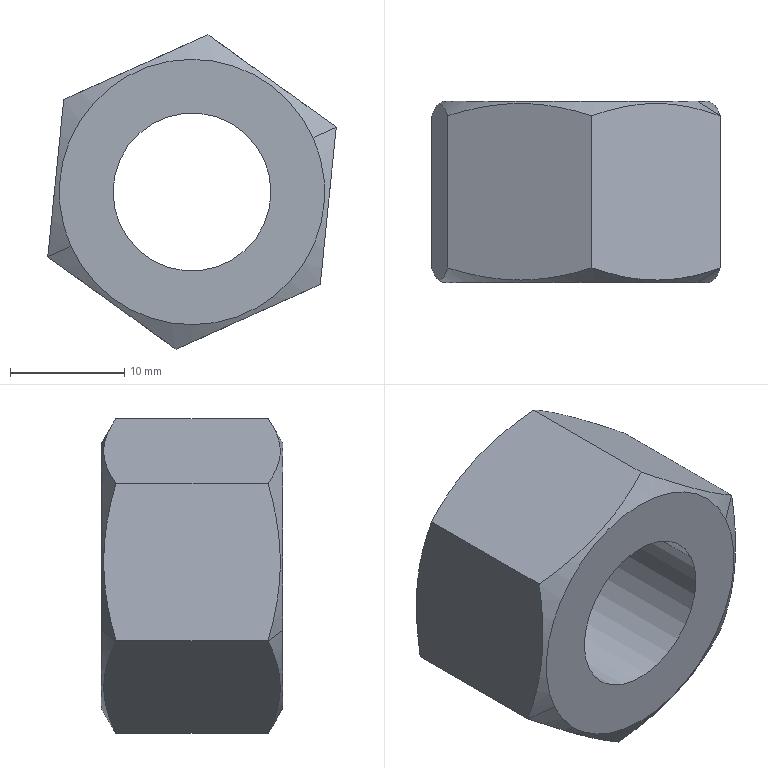Component | SolidWorks | YC1-250-04BalancerAssembly#16673-1_GBHexNutM20_GB_FASTENER_NUT_SNC1M16-N-1 | 1 solid | 14 faces | box 25.28 x 15.9 x 27.57 mm | volume 5485 mm3 | plane 8 | cone 4 | cylinder 2 | commonest cylinder face diameters 13.835 x2 | material Plain Carbon Steel
STEP:
#1=COLOUR_RGB('',0.7922,0.8196,0.9333);
#2=FILL_AREA_STYLE_COLOUR('',#1);
#3=FILL_AREA_STYLE('',(#2));
#4=SURFACE_STYLE_FILL_AREA(#3);
#5=SURFACE_SIDE_STYLE('',(#4));
#6=SURFACE_STYLE_USAGE(.BOTH.,#5);
#7=PRESENTATION_STYLE_ASSIGNMENT((#6));
#8=CARTESIAN_POINT('',(-13.129,180.709,-4.621));
#9=VERTEX_POINT('',#8);
#10=CARTESIAN_POINT('',(-13.626,180.709,-4.844));
#11=VERTEX_POINT('',#10);
#12=CARTESIAN_POINT('',(-13.378,180.709,-4.733));
#13=DIRECTION('',(-0.,-1.,0.));
#14=DIRECTION('',(-0.9121,0.,-0.41));
#15=AXIS2_PLACEMENT_3D('',#12,#13,#14);
#16=CIRCLE('',#15,0.2723);
#17=EDGE_CURVE('',#9,#11,#16,.T.);
#18=ORIENTED_EDGE('',*,*,#17,.F.);
#19=CARTESIAN_POINT('',(-13.129,180.083,-4.621));
#20=VERTEX_POINT('',#19);
#21=CARTESIAN_POINT('',(-13.129,180.709,-4.621));
#22=DIRECTION('',(-0.,-1.,0.));
#23=VECTOR('',#22,39.37);
#24=LINE('',#21,#23);
#25=EDGE_CURVE('',#9,#20,#24,.T.);
#26=ORIENTED_EDGE('',*,*,#25,.T.);
#27=CARTESIAN_POINT('',(-13.626,180.083,-4.844));
#28=VERTEX_POINT('',#27);
#29=CARTESIAN_POINT('',(-13.378,180.083,-4.733));
#30=DIRECTION('',(0.,1.,-0.));
#31=DIRECTION('',(-0.9121,0.,-0.41));
#32=AXIS2_PLACEMENT_3D('',#29,#30,#31);
#33=CIRCLE('',#32,0.2723);
#34=EDGE_CURVE('',#28,#20,#33,.T.);
#35=ORIENTED_EDGE('',*,*,#34,.F.);
#36=CARTESIAN_POINT('',(-13.626,180.709,-4.844));
#37=DIRECTION('',(-0.,-1.,0.));
#38=VECTOR('',#37,39.37);
#39=LINE('',#36,#38);
#40=EDGE_CURVE('',#11,#28,#39,.T.);
#41=ORIENTED_EDGE('',*,*,#40,.F.);
#42=EDGE_LOOP('',(#18,#26,#35,#41));
#43=FACE_OUTER_BOUND('',#42,.T.);
#44=CARTESIAN_POINT('',(-13.378,180.709,-4.733));
#45=DIRECTION('',(-0.,-1.,0.));
#46=DIRECTION('',(-0.9121,0.,-0.41));
#47=AXIS2_PLACEMENT_3D('',#44,#45,#46);
#48=CYLINDRICAL_SURFACE('',#47,0.2723);
#49=ADVANCED_FACE('',(#43),#48,.F.);
#50=CARTESIAN_POINT('',(-13.795,180.709,-4.92));
#51=VERTEX_POINT('',#50);
#52=CARTESIAN_POINT('',(-12.96,180.709,-4.545));
#53=VERTEX_POINT('',#52);
#54=CARTESIAN_POINT('',(-13.378,180.709,-4.733));
#55=DIRECTION('',(-0.,-1.,0.));
#56=DIRECTION('',(-0.9121,0.,-0.41));
#57=AXIS2_PLACEMENT_3D('',#54,#55,#56);
#58=CIRCLE('',#57,0.4577);
#59=EDGE_CURVE('',#51,#53,#58,.T.);
#60=ORIENTED_EDGE('',*,*,#59,.T.);
#61=CARTESIAN_POINT('',(-12.88,180.658,-4.509));
#62=VERTEX_POINT('',#61);
#63=CARTESIAN_POINT('',(-12.88,180.658,-4.509));
#64=DIRECTION('',(0.7899,-0.5,0.3551));
#65=VECTOR('',#64,39.37);
#66=LINE('',#63,#65);
#67=EDGE_CURVE('',#53,#62,#66,.T.);
#68=ORIENTED_EDGE('',*,*,#67,.T.);
#69=CARTESIAN_POINT('',(-12.935,180.658,-5.052));
#70=VERTEX_POINT('',#69);
#71=CARTESIAN_POINT('',(-12.88,180.658,-4.509));
#72=CARTESIAN_POINT('',(-12.885,180.671,-4.553));
#73=CARTESIAN_POINT('',(-12.889,180.681,-4.598));
#74=CARTESIAN_POINT('',(-12.898,180.696,-4.688));
#75=CARTESIAN_POINT('',(-12.903,180.7,-4.734));
#76=CARTESIAN_POINT('',(-12.91,180.7,-4.803));
#77=CARTESIAN_POINT('',(-12.912,180.699,-4.826));
#78=CARTESIAN_POINT('',(-12.917,180.695,-4.872));
#79=CARTESIAN_POINT('',(-12.919,180.692,-4.895));
#80=CARTESIAN_POINT('',(-12.926,180.681,-4.963));
#81=CARTESIAN_POINT('',(-12.931,180.671,-5.007));
#82=CARTESIAN_POINT('',(-12.935,180.658,-5.052));
#83=B_SPLINE_CURVE_WITH_KNOTS('',3,(#71,#72,#73,#74,#75,#76,#77,#78,#79,#80,#81,#82),.UNSPECIFIED.,.F.,.F.,(4,2,2,2,2,4),(0.,0.003499,0.006997,0.008746,0.0105,0.01399),.UNSPECIFIED.);
#84=EDGE_CURVE('',#62,#70,#83,.T.);
#85=ORIENTED_EDGE('',*,*,#84,.T.);
#86=CARTESIAN_POINT('',(-13.433,180.658,-5.275));
#87=VERTEX_POINT('',#86);
#88=CARTESIAN_POINT('',(-12.935,180.658,-5.052));
#89=CARTESIAN_POINT('',(-12.976,180.671,-5.07));
#90=CARTESIAN_POINT('',(-13.017,180.681,-5.088));
#91=CARTESIAN_POINT('',(-13.099,180.696,-5.125));
#92=CARTESIAN_POINT('',(-13.141,180.7,-5.144));
#93=CARTESIAN_POINT('',(-13.205,180.7,-5.173));
#94=CARTESIAN_POINT('',(-13.226,180.699,-5.182));
#95=CARTESIAN_POINT('',(-13.268,180.695,-5.201));
#96=CARTESIAN_POINT('',(-13.289,180.692,-5.211));
#97=CARTESIAN_POINT('',(-13.351,180.681,-5.239));
#98=CARTESIAN_POINT('',(-13.392,180.671,-5.257));
#99=CARTESIAN_POINT('',(-13.433,180.658,-5.275));
#100=B_SPLINE_CURVE_WITH_KNOTS('',3,(#88,#89,#90,#91,#92,#93,#94,#95,#96,#97,#98,#99),.UNSPECIFIED.,.F.,.F.,(4,2,2,2,2,4),(0.,0.003499,0.006997,0.008746,0.0105,0.01399),.UNSPECIFIED.);
#101=EDGE_CURVE('',#70,#87,#100,.T.);
#102=ORIENTED_EDGE('',*,*,#101,.T.);
#103=CARTESIAN_POINT('',(-13.875,180.658,-4.956));
#104=VERTEX_POINT('',#103);
#105=CARTESIAN_POINT('',(-13.433,180.658,-5.275));
#106=CARTESIAN_POINT('',(-13.469,180.671,-5.249));
#107=CARTESIAN_POINT('',(-13.505,180.681,-5.223));
#108=CARTESIAN_POINT('',(-13.579,180.696,-5.17));
#109=CARTESIAN_POINT('',(-13.616,180.7,-5.143));
#110=CARTESIAN_POINT('',(-13.672,180.7,-5.103));
#111=CARTESIAN_POINT('',(-13.691,180.699,-5.089));
#112=CARTESIAN_POINT('',(-13.729,180.695,-5.062));
#113=CARTESIAN_POINT('',(-13.747,180.692,-5.049));
#114=CARTESIAN_POINT('',(-13.803,180.681,-5.009));
#115=CARTESIAN_POINT('',(-13.839,180.671,-4.982));
#116=CARTESIAN_POINT('',(-13.875,180.658,-4.956));
#117=B_SPLINE_CURVE_WITH_KNOTS('',3,(#105,#106,#107,#108,#109,#110,#111,#112,#113,#114,#115,#116),.UNSPECIFIED.,.F.,.F.,(4,2,2,2,2,4),(0.,0.003499,0.006997,0.008746,0.0105,0.01399),.UNSPECIFIED.);
#118=EDGE_CURVE('',#87,#104,#117,.T.);
#119=ORIENTED_EDGE('',*,*,#118,.T.);
#120=CARTESIAN_POINT('',(-13.876,180.658,-4.957));
#121=DIRECTION('',(-0.7899,-0.5,-0.3551));
#122=VECTOR('',#121,39.37);
#123=LINE('',#120,#122);
#124=EDGE_CURVE('',#51,#104,#123,.T.);
#125=ORIENTED_EDGE('',*,*,#124,.F.);
#126=EDGE_LOOP('',(#60,#68,#85,#102,#119,#125));
#127=FACE_OUTER_BOUND('',#126,.T.);
#128=CARTESIAN_POINT('',(-13.378,180.658,-4.733));
#129=DIRECTION('',(-0.,-1.,0.));
#130=DIRECTION('',(-0.9121,0.,-0.41));
#131=AXIS2_PLACEMENT_3D('',#128,#129,#130);
#132=CONICAL_SURFACE('',#131,0.5461,1.047);
#133=ADVANCED_FACE('',(#127),#132,.T.);
#134=CARTESIAN_POINT('',(-13.795,180.083,-4.92));
#135=VERTEX_POINT('',#134);
#136=CARTESIAN_POINT('',(-12.96,180.083,-4.545));
#137=VERTEX_POINT('',#136);
#138=CARTESIAN_POINT('',(-13.378,180.083,-4.733));
#139=DIRECTION('',(-0.,-1.,0.));
#140=DIRECTION('',(0.9121,0.,0.41));
#141=AXIS2_PLACEMENT_3D('',#138,#139,#140);
#142=CIRCLE('',#141,0.4577);
#143=EDGE_CURVE('',#135,#137,#142,.T.);
#144=ORIENTED_EDGE('',*,*,#143,.F.);
#145=CARTESIAN_POINT('',(-13.875,180.133,-4.956));
#146=VERTEX_POINT('',#145);
#147=CARTESIAN_POINT('',(-13.876,180.134,-4.957));
#148=DIRECTION('',(-0.7899,0.5,-0.3551));
#149=VECTOR('',#148,39.37);
#150=LINE('',#147,#149);
#151=EDGE_CURVE('',#135,#146,#150,.T.);
#152=ORIENTED_EDGE('',*,*,#151,.T.);
#153=CARTESIAN_POINT('',(-13.433,180.133,-5.275));
#154=VERTEX_POINT('',#153);
#155=CARTESIAN_POINT('',(-13.875,180.133,-4.956));
#156=CARTESIAN_POINT('',(-13.839,180.121,-4.982));
#157=CARTESIAN_POINT('',(-13.803,180.11,-5.009));
#158=CARTESIAN_POINT('',(-13.729,180.095,-5.062));
#159=CARTESIAN_POINT('',(-13.692,180.091,-5.088));
#160=CARTESIAN_POINT('',(-13.636,180.091,-5.129));
#161=CARTESIAN_POINT('',(-13.617,180.092,-5.143));
#162=CARTESIAN_POINT('',(-13.579,180.096,-5.17));
#163=CARTESIAN_POINT('',(-13.561,180.099,-5.183));
#164=CARTESIAN_POINT('',(-13.505,180.11,-5.223));
#165=CARTESIAN_POINT('',(-13.469,180.121,-5.249));
#166=CARTESIAN_POINT('',(-13.433,180.133,-5.275));
#167=B_SPLINE_CURVE_WITH_KNOTS('',3,(#155,#156,#157,#158,#159,#160,#161,#162,#163,#164,#165,#166),.UNSPECIFIED.,.F.,.F.,(4,2,2,2,2,4),(0.,0.003499,0.006997,0.008746,0.0105,0.01399),.UNSPECIFIED.);
#168=EDGE_CURVE('',#146,#154,#167,.T.);
#169=ORIENTED_EDGE('',*,*,#168,.T.);
#170=CARTESIAN_POINT('',(-12.935,180.133,-5.052));
#171=VERTEX_POINT('',#170);
#172=CARTESIAN_POINT('',(-13.433,180.133,-5.275));
#173=CARTESIAN_POINT('',(-13.392,180.121,-5.257));
#174=CARTESIAN_POINT('',(-13.351,180.11,-5.239));
#175=CARTESIAN_POINT('',(-13.268,180.095,-5.202));
#176=CARTESIAN_POINT('',(-13.227,180.091,-5.183));
#177=CARTESIAN_POINT('',(-13.163,180.091,-5.154));
#178=CARTESIAN_POINT('',(-13.142,180.092,-5.145));
#179=CARTESIAN_POINT('',(-13.1,180.096,-5.126));
#180=CARTESIAN_POINT('',(-13.079,180.099,-5.116));
#181=CARTESIAN_POINT('',(-13.017,180.11,-5.088));
#182=CARTESIAN_POINT('',(-12.976,180.121,-5.07));
#183=CARTESIAN_POINT('',(-12.935,180.133,-5.052));
#184=B_SPLINE_CURVE_WITH_KNOTS('',3,(#172,#173,#174,#175,#176,#177,#178,#179,#180,#181,#182,#183),.UNSPECIFIED.,.F.,.F.,(4,2,2,2,2,4),(0.,0.003499,0.006997,0.008746,0.0105,0.01399),.UNSPECIFIED.);
#185=EDGE_CURVE('',#154,#171,#184,.T.);
#186=ORIENTED_EDGE('',*,*,#185,.T.);
#187=CARTESIAN_POINT('',(-12.88,180.133,-4.509));
#188=VERTEX_POINT('',#187);
#189=CARTESIAN_POINT('',(-12.935,180.133,-5.052));
#190=CARTESIAN_POINT('',(-12.931,180.121,-5.007));
#191=CARTESIAN_POINT('',(-12.926,180.11,-4.963));
#192=CARTESIAN_POINT('',(-12.917,180.095,-4.873));
#193=CARTESIAN_POINT('',(-12.912,180.091,-4.827));
#194=CARTESIAN_POINT('',(-12.905,180.091,-4.758));
#195=CARTESIAN_POINT('',(-12.903,180.092,-4.735));
#196=CARTESIAN_POINT('',(-12.898,180.096,-4.689));
#197=CARTESIAN_POINT('',(-12.896,180.099,-4.666));
#198=CARTESIAN_POINT('',(-12.889,180.11,-4.598));
#199=CARTESIAN_POINT('',(-12.885,180.121,-4.553));
#200=CARTESIAN_POINT('',(-12.88,180.133,-4.509));
#201=B_SPLINE_CURVE_WITH_KNOTS('',3,(#189,#190,#191,#192,#193,#194,#195,#196,#197,#198,#199,#200),.UNSPECIFIED.,.F.,.F.,(4,2,2,2,2,4),(0.,0.003499,0.006997,0.008746,0.0105,0.01399),.UNSPECIFIED.);
#202=EDGE_CURVE('',#171,#188,#201,.T.);
#203=ORIENTED_EDGE('',*,*,#202,.T.);
#204=CARTESIAN_POINT('',(-12.88,180.134,-4.509));
#205=DIRECTION('',(0.7899,0.5,0.3551));
#206=VECTOR('',#205,39.37);
#207=LINE('',#204,#206);
#208=EDGE_CURVE('',#137,#188,#207,.T.);
#209=ORIENTED_EDGE('',*,*,#208,.F.);
#210=EDGE_LOOP('',(#144,#152,#169,#186,#203,#209));
#211=FACE_OUTER_BOUND('',#210,.T.);
#212=CARTESIAN_POINT('',(-13.378,180.134,-4.733));
#213=DIRECTION('',(0.,1.,-0.));
#214=DIRECTION('',(0.9121,0.,0.41));
#215=AXIS2_PLACEMENT_3D('',#212,#213,#214);
#216=CONICAL_SURFACE('',#215,0.5461,1.047);
#217=ADVANCED_FACE('',(#211),#216,.T.);
#218=ORIENTED_EDGE('',*,*,#25,.F.);
#219=CARTESIAN_POINT('',(-13.378,180.709,-4.733));
#220=DIRECTION('',(-0.,-1.,0.));
#221=DIRECTION('',(-0.9121,0.,-0.41));
#222=AXIS2_PLACEMENT_3D('',#219,#220,#221);
#223=CIRCLE('',#222,0.2723);
#224=EDGE_CURVE('',#11,#9,#223,.T.);
#225=ORIENTED_EDGE('',*,*,#224,.F.);
#226=ORIENTED_EDGE('',*,*,#40,.T.);
#227=CARTESIAN_POINT('',(-13.378,180.083,-4.733));
#228=DIRECTION('',(0.,1.,-0.));
#229=DIRECTION('',(-0.9121,0.,-0.41));
#230=AXIS2_PLACEMENT_3D('',#227,#228,#229);
#231=CIRCLE('',#230,0.2723);
#232=EDGE_CURVE('',#20,#28,#231,.T.);
#233=ORIENTED_EDGE('',*,*,#232,.F.);
#234=EDGE_LOOP('',(#218,#225,#226,#233));
#235=FACE_OUTER_BOUND('',#234,.T.);
#236=CARTESIAN_POINT('',(-13.378,180.709,-4.733));
#237=DIRECTION('',(-0.,-1.,0.));
#238=DIRECTION('',(-0.9121,0.,-0.41));
#239=AXIS2_PLACEMENT_3D('',#236,#237,#238);
#240=CYLINDRICAL_SURFACE('',#239,0.2723);
#241=ADVANCED_FACE('',(#235),#240,.F.);
#242=ORIENTED_EDGE('',*,*,#224,.T.);
#243=ORIENTED_EDGE('',*,*,#17,.T.);
#244=EDGE_LOOP('',(#242,#243));
#245=FACE_BOUND('',#244,.T.);
#246=ORIENTED_EDGE('',*,*,#59,.F.);
#247=CARTESIAN_POINT('',(-13.378,180.709,-4.733));
#248=DIRECTION('',(-0.,-1.,0.));
#249=DIRECTION('',(-0.9121,0.,-0.41));
#250=AXIS2_PLACEMENT_3D('',#247,#248,#249);
#251=CIRCLE('',#250,0.4577);
#252=EDGE_CURVE('',#53,#51,#251,.T.);
#253=ORIENTED_EDGE('',*,*,#252,.F.);
#254=EDGE_LOOP('',(#246,#253));
#255=FACE_OUTER_BOUND('',#254,.T.);
#256=CARTESIAN_POINT('',(-13.82,180.709,-4.414));
#257=DIRECTION('',(-0.,-1.,0.));
#258=DIRECTION('',(-0.9121,-0.,-0.41));
#259=AXIS2_PLACEMENT_3D('',#256,#257,#258);
#260=PLANE('',#259);
#261=ADVANCED_FACE('',(#245,#255),#260,.F.);
#262=ORIENTED_EDGE('',*,*,#34,.T.);
#263=ORIENTED_EDGE('',*,*,#232,.T.);
#264=EDGE_LOOP('',(#262,#263));
#265=FACE_BOUND('',#264,.T.);
#266=CARTESIAN_POINT('',(-13.378,180.083,-4.733));
#267=DIRECTION('',(-0.,-1.,0.));
#268=DIRECTION('',(0.9121,0.,0.41));
#269=AXIS2_PLACEMENT_3D('',#266,#267,#268);
#270=CIRCLE('',#269,0.4577);
#271=EDGE_CURVE('',#137,#135,#270,.T.);
#272=ORIENTED_EDGE('',*,*,#271,.T.);
#273=ORIENTED_EDGE('',*,*,#143,.T.);
#274=EDGE_LOOP('',(#272,#273));
#275=FACE_OUTER_BOUND('',#274,.T.);
#276=CARTESIAN_POINT('',(-13.82,180.083,-4.414));
#277=DIRECTION('',(-0.,-1.,0.));
#278=DIRECTION('',(-0.9121,-0.,-0.41));
#279=AXIS2_PLACEMENT_3D('',#276,#277,#278);
#280=PLANE('',#279);
#281=ADVANCED_FACE('',(#265,#275),#280,.T.);
#282=ORIENTED_EDGE('',*,*,#67,.F.);
#283=ORIENTED_EDGE('',*,*,#252,.T.);
#284=ORIENTED_EDGE('',*,*,#124,.T.);
#285=CARTESIAN_POINT('',(-13.82,180.658,-4.414));
#286=VERTEX_POINT('',#285);
#287=CARTESIAN_POINT('',(-13.875,180.658,-4.956));
#288=CARTESIAN_POINT('',(-13.871,180.671,-4.912));
#289=CARTESIAN_POINT('',(-13.866,180.681,-4.867));
#290=CARTESIAN_POINT('',(-13.857,180.696,-4.777));
#291=CARTESIAN_POINT('',(-13.852,180.7,-4.732));
#292=CARTESIAN_POINT('',(-13.845,180.7,-4.662));
#293=CARTESIAN_POINT('',(-13.843,180.699,-4.639));
#294=CARTESIAN_POINT('',(-13.838,180.695,-4.593));
#295=CARTESIAN_POINT('',(-13.836,180.692,-4.571));
#296=CARTESIAN_POINT('',(-13.829,180.681,-4.503));
#297=CARTESIAN_POINT('',(-13.825,180.671,-4.458));
#298=CARTESIAN_POINT('',(-13.82,180.658,-4.414));
#299=B_SPLINE_CURVE_WITH_KNOTS('',3,(#287,#288,#289,#290,#291,#292,#293,#294,#295,#296,#297,#298),.UNSPECIFIED.,.F.,.F.,(4,2,2,2,2,4),(0.,0.003499,0.006997,0.008746,0.0105,0.01399),.UNSPECIFIED.);
#300=EDGE_CURVE('',#104,#286,#299,.T.);
#301=ORIENTED_EDGE('',*,*,#300,.T.);
#302=CARTESIAN_POINT('',(-13.323,180.658,-4.19));
#303=VERTEX_POINT('',#302);
#304=CARTESIAN_POINT('',(-13.82,180.658,-4.414));
#305=CARTESIAN_POINT('',(-13.78,180.671,-4.395));
#306=CARTESIAN_POINT('',(-13.739,180.681,-4.377));
#307=CARTESIAN_POINT('',(-13.656,180.696,-4.34));
#308=CARTESIAN_POINT('',(-13.614,180.7,-4.321));
#309=CARTESIAN_POINT('',(-13.551,180.7,-4.292));
#310=CARTESIAN_POINT('',(-13.529,180.699,-4.283));
#311=CARTESIAN_POINT('',(-13.487,180.695,-4.264));
#312=CARTESIAN_POINT('',(-13.467,180.692,-4.255));
#313=CARTESIAN_POINT('',(-13.404,180.681,-4.227));
#314=CARTESIAN_POINT('',(-13.363,180.671,-4.208));
#315=CARTESIAN_POINT('',(-13.323,180.658,-4.19));
#316=B_SPLINE_CURVE_WITH_KNOTS('',3,(#304,#305,#306,#307,#308,#309,#310,#311,#312,#313,#314,#315),.UNSPECIFIED.,.F.,.F.,(4,2,2,2,2,4),(0.,0.003499,0.006997,0.008746,0.0105,0.01399),.UNSPECIFIED.);
#317=EDGE_CURVE('',#286,#303,#316,.T.);
#318=ORIENTED_EDGE('',*,*,#317,.T.);
#319=CARTESIAN_POINT('',(-13.323,180.658,-4.19));
#320=CARTESIAN_POINT('',(-13.286,180.671,-4.216));
#321=CARTESIAN_POINT('',(-13.25,180.681,-4.242));
#322=CARTESIAN_POINT('',(-13.177,180.696,-4.295));
#323=CARTESIAN_POINT('',(-13.139,180.7,-4.322));
#324=CARTESIAN_POINT('',(-13.083,180.7,-4.363));
#325=CARTESIAN_POINT('',(-13.064,180.699,-4.376));
#326=CARTESIAN_POINT('',(-13.027,180.695,-4.403));
#327=CARTESIAN_POINT('',(-13.008,180.692,-4.417));
#328=CARTESIAN_POINT('',(-12.953,180.681,-4.457));
#329=CARTESIAN_POINT('',(-12.916,180.671,-4.483));
#330=CARTESIAN_POINT('',(-12.88,180.658,-4.509));
#331=B_SPLINE_CURVE_WITH_KNOTS('',3,(#319,#320,#321,#322,#323,#324,#325,#326,#327,#328,#329,#330),.UNSPECIFIED.,.F.,.F.,(4,2,2,2,2,4),(0.,0.003499,0.006997,0.008746,0.0105,0.01399),.UNSPECIFIED.);
#332=EDGE_CURVE('',#303,#62,#331,.T.);
#333=ORIENTED_EDGE('',*,*,#332,.T.);
#334=EDGE_LOOP('',(#282,#283,#284,#301,#318,#333));
#335=FACE_OUTER_BOUND('',#334,.T.);
#336=CARTESIAN_POINT('',(-13.378,180.658,-4.733));
#337=DIRECTION('',(-0.,-1.,0.));
#338=DIRECTION('',(-0.9121,0.,-0.41));
#339=AXIS2_PLACEMENT_3D('',#336,#337,#338);
#340=CONICAL_SURFACE('',#339,0.5461,1.047);
#341=ADVANCED_FACE('',(#335),#340,.T.);
#342=ORIENTED_EDGE('',*,*,#151,.F.);
#343=ORIENTED_EDGE('',*,*,#271,.F.);
#344=ORIENTED_EDGE('',*,*,#208,.T.);
#345=CARTESIAN_POINT('',(-13.323,180.133,-4.19));
#346=VERTEX_POINT('',#345);
#347=CARTESIAN_POINT('',(-12.88,180.133,-4.509));
#348=CARTESIAN_POINT('',(-12.916,180.121,-4.483));
#349=CARTESIAN_POINT('',(-12.953,180.11,-4.457));
#350=CARTESIAN_POINT('',(-13.026,180.095,-4.404));
#351=CARTESIAN_POINT('',(-13.063,180.091,-4.377));
#352=CARTESIAN_POINT('',(-13.12,180.091,-4.336));
#353=CARTESIAN_POINT('',(-13.139,180.092,-4.323));
#354=CARTESIAN_POINT('',(-13.176,180.096,-4.296));
#355=CARTESIAN_POINT('',(-13.195,180.099,-4.282));
#356=CARTESIAN_POINT('',(-13.25,180.11,-4.242));
#357=CARTESIAN_POINT('',(-13.286,180.121,-4.216));
#358=CARTESIAN_POINT('',(-13.323,180.133,-4.19));
#359=B_SPLINE_CURVE_WITH_KNOTS('',3,(#347,#348,#349,#350,#351,#352,#353,#354,#355,#356,#357,#358),.UNSPECIFIED.,.F.,.F.,(4,2,2,2,2,4),(0.,0.003499,0.006997,0.008746,0.0105,0.01399),.UNSPECIFIED.);
#360=EDGE_CURVE('',#188,#346,#359,.T.);
#361=ORIENTED_EDGE('',*,*,#360,.T.);
#362=CARTESIAN_POINT('',(-13.82,180.133,-4.414));
#363=VERTEX_POINT('',#362);
#364=CARTESIAN_POINT('',(-13.323,180.133,-4.19));
#365=CARTESIAN_POINT('',(-13.363,180.121,-4.208));
#366=CARTESIAN_POINT('',(-13.404,180.11,-4.227));
#367=CARTESIAN_POINT('',(-13.487,180.095,-4.264));
#368=CARTESIAN_POINT('',(-13.529,180.091,-4.282));
#369=CARTESIAN_POINT('',(-13.592,180.091,-4.311));
#370=CARTESIAN_POINT('',(-13.613,180.092,-4.321));
#371=CARTESIAN_POINT('',(-13.655,180.096,-4.339));
#372=CARTESIAN_POINT('',(-13.676,180.099,-4.349));
#373=CARTESIAN_POINT('',(-13.738,180.11,-4.377));
#374=CARTESIAN_POINT('',(-13.779,180.121,-4.395));
#375=CARTESIAN_POINT('',(-13.82,180.133,-4.414));
#376=B_SPLINE_CURVE_WITH_KNOTS('',3,(#364,#365,#366,#367,#368,#369,#370,#371,#372,#373,#374,#375),.UNSPECIFIED.,.F.,.F.,(4,2,2,2,2,4),(0.,0.003499,0.006997,0.008746,0.0105,0.01399),.UNSPECIFIED.);
#377=EDGE_CURVE('',#346,#363,#376,.T.);
#378=ORIENTED_EDGE('',*,*,#377,.T.);
#379=CARTESIAN_POINT('',(-13.82,180.133,-4.414));
#380=CARTESIAN_POINT('',(-13.825,180.121,-4.458));
#381=CARTESIAN_POINT('',(-13.829,180.11,-4.502));
#382=CARTESIAN_POINT('',(-13.838,180.095,-4.593));
#383=CARTESIAN_POINT('',(-13.843,180.091,-4.638));
#384=CARTESIAN_POINT('',(-13.85,180.091,-4.707));
#385=CARTESIAN_POINT('',(-13.852,180.092,-4.731));
#386=CARTESIAN_POINT('',(-13.857,180.096,-4.777));
#387=CARTESIAN_POINT('',(-13.859,180.099,-4.799));
#388=CARTESIAN_POINT('',(-13.866,180.11,-4.867));
#389=CARTESIAN_POINT('',(-13.871,180.121,-4.912));
#390=CARTESIAN_POINT('',(-13.875,180.133,-4.956));
#391=B_SPLINE_CURVE_WITH_KNOTS('',3,(#379,#380,#381,#382,#383,#384,#385,#386,#387,#388,#389,#390),.UNSPECIFIED.,.F.,.F.,(4,2,2,2,2,4),(0.,0.003499,0.006997,0.008746,0.0105,0.01399),.UNSPECIFIED.);
#392=EDGE_CURVE('',#363,#146,#391,.T.);
#393=ORIENTED_EDGE('',*,*,#392,.T.);
#394=EDGE_LOOP('',(#342,#343,#344,#361,#378,#393));
#395=FACE_OUTER_BOUND('',#394,.T.);
#396=CARTESIAN_POINT('',(-13.378,180.134,-4.733));
#397=DIRECTION('',(0.,1.,-0.));
#398=DIRECTION('',(0.9121,0.,0.41));
#399=AXIS2_PLACEMENT_3D('',#396,#397,#398);
#400=CONICAL_SURFACE('',#399,0.5461,1.047);
#401=ADVANCED_FACE('',(#395),#400,.T.);
#402=ORIENTED_EDGE('',*,*,#332,.F.);
#403=CARTESIAN_POINT('',(-13.323,180.709,-4.19));
#404=DIRECTION('',(-0.,-1.,0.));
#405=VECTOR('',#404,39.37);
#406=LINE('',#403,#405);
#407=EDGE_CURVE('',#303,#346,#406,.T.);
#408=ORIENTED_EDGE('',*,*,#407,.T.);
#409=ORIENTED_EDGE('',*,*,#360,.F.);
#410=CARTESIAN_POINT('',(-12.88,180.709,-4.509));
#411=DIRECTION('',(0.,1.,-0.));
#412=VECTOR('',#411,39.37);
#413=LINE('',#410,#412);
#414=EDGE_CURVE('',#188,#62,#413,.T.);
#415=ORIENTED_EDGE('',*,*,#414,.T.);
#416=EDGE_LOOP('',(#402,#408,#409,#415));
#417=FACE_OUTER_BOUND('',#416,.T.);
#418=CARTESIAN_POINT('',(-12.88,180.709,-4.509));
#419=DIRECTION('',(0.5848,0.,0.8111));
#420=DIRECTION('',(-0.8111,0.,0.5848));
#421=AXIS2_PLACEMENT_3D('',#418,#419,#420);
#422=PLANE('',#421);
#423=ADVANCED_FACE('',(#417),#422,.T.);
#424=ORIENTED_EDGE('',*,*,#317,.F.);
#425=CARTESIAN_POINT('',(-13.82,180.709,-4.414));
#426=DIRECTION('',(-0.,-1.,0.));
#427=VECTOR('',#426,39.37);
#428=LINE('',#425,#427);
#429=EDGE_CURVE('',#286,#363,#428,.T.);
#430=ORIENTED_EDGE('',*,*,#429,.T.);
#431=ORIENTED_EDGE('',*,*,#377,.F.);
#432=ORIENTED_EDGE('',*,*,#407,.F.);
#433=EDGE_LOOP('',(#424,#430,#431,#432));
#434=FACE_OUTER_BOUND('',#433,.T.);
#435=CARTESIAN_POINT('',(-13.323,180.709,-4.19));
#436=DIRECTION('',(-0.41,0.,0.9121));
#437=DIRECTION('',(-0.9121,-0.,-0.41));
#438=AXIS2_PLACEMENT_3D('',#435,#436,#437);
#439=PLANE('',#438);
#440=ADVANCED_FACE('',(#434),#439,.T.);
#441=ORIENTED_EDGE('',*,*,#300,.F.);
#442=CARTESIAN_POINT('',(-13.875,180.709,-4.956));
#443=DIRECTION('',(-0.,-1.,0.));
#444=VECTOR('',#443,39.37);
#445=LINE('',#442,#444);
#446=EDGE_CURVE('',#104,#146,#445,.T.);
#447=ORIENTED_EDGE('',*,*,#446,.T.);
#448=ORIENTED_EDGE('',*,*,#392,.F.);
#449=ORIENTED_EDGE('',*,*,#429,.F.);
#450=EDGE_LOOP('',(#441,#447,#448,#449));
#451=FACE_OUTER_BOUND('',#450,.T.);
#452=CARTESIAN_POINT('',(-13.82,180.709,-4.414));
#453=DIRECTION('',(-0.9949,0.,0.1009));
#454=DIRECTION('',(-0.1009,-0.,-0.9949));
#455=AXIS2_PLACEMENT_3D('',#452,#453,#454);
#456=PLANE('',#455);
#457=ADVANCED_FACE('',(#451),#456,.T.);
#458=ORIENTED_EDGE('',*,*,#118,.F.);
#459=CARTESIAN_POINT('',(-13.433,180.709,-5.275));
#460=DIRECTION('',(-0.,-1.,0.));
#461=VECTOR('',#460,39.37);
#462=LINE('',#459,#461);
#463=EDGE_CURVE('',#87,#154,#462,.T.);
#464=ORIENTED_EDGE('',*,*,#463,.T.);
#465=ORIENTED_EDGE('',*,*,#168,.F.);
#466=ORIENTED_EDGE('',*,*,#446,.F.);
#467=EDGE_LOOP('',(#458,#464,#465,#466));
#468=FACE_OUTER_BOUND('',#467,.T.);
#469=CARTESIAN_POINT('',(-13.875,180.709,-4.956));
#470=DIRECTION('',(-0.5848,-0.,-0.8111));
#471=DIRECTION('',(0.8111,-0.,-0.5848));
#472=AXIS2_PLACEMENT_3D('',#469,#470,#471);
#473=PLANE('',#472);
#474=ADVANCED_FACE('',(#468),#473,.T.);
#475=ORIENTED_EDGE('',*,*,#101,.F.);
#476=CARTESIAN_POINT('',(-12.935,180.709,-5.052));
#477=DIRECTION('',(-0.,-1.,0.));
#478=VECTOR('',#477,39.37);
#479=LINE('',#476,#478);
#480=EDGE_CURVE('',#70,#171,#479,.T.);
#481=ORIENTED_EDGE('',*,*,#480,.T.);
#482=ORIENTED_EDGE('',*,*,#185,.F.);
#483=ORIENTED_EDGE('',*,*,#463,.F.);
#484=EDGE_LOOP('',(#475,#481,#482,#483));
#485=FACE_OUTER_BOUND('',#484,.T.);
#486=CARTESIAN_POINT('',(-13.433,180.709,-5.275));
#487=DIRECTION('',(0.41,-0.,-0.9121));
#488=DIRECTION('',(-0.,-1.,0.));
#489=AXIS2_PLACEMENT_3D('',#486,#487,#488);
#490=PLANE('',#489);
#491=ADVANCED_FACE('',(#485),#490,.T.);
#492=ORIENTED_EDGE('',*,*,#84,.F.);
#493=ORIENTED_EDGE('',*,*,#414,.F.);
#494=ORIENTED_EDGE('',*,*,#202,.F.);
#495=ORIENTED_EDGE('',*,*,#480,.F.);
#496=EDGE_LOOP('',(#492,#493,#494,#495));
#497=FACE_OUTER_BOUND('',#496,.T.);
#498=CARTESIAN_POINT('',(-12.935,180.709,-5.052));
#499=DIRECTION('',(0.9949,-0.,-0.1009));
#500=DIRECTION('',(0.1009,0.,0.9949));
#501=AXIS2_PLACEMENT_3D('',#498,#499,#500);
#502=PLANE('',#501);
#503=ADVANCED_FACE('',(#497),#502,.T.);
#504=CLOSED_SHELL('',(#49,#133,#217,#241,#261,#281,#341,#401,#423,#440,#457,#474,#491,#503));
#505=MANIFOLD_SOLID_BREP('',#504);
#506=STYLED_ITEM('',(#7),#505);
#507=(LENGTH_UNIT()NAMED_UNIT(*)SI_UNIT($,.METRE.));
#508=LENGTH_MEASURE_WITH_UNIT(LENGTH_MEASURE(0.0254),#507);
#509=DIMENSIONAL_EXPONENTS(1.,0.,0.,0.,0.,0.,0.);
#510=(CONVERSION_BASED_UNIT('',#508)LENGTH_UNIT()NAMED_UNIT(#509));
#511=UNCERTAINTY_MEASURE_WITH_UNIT(LENGTH_MEASURE(0.00001),#510,'','');
#512=(NAMED_UNIT(*)PLANE_ANGLE_UNIT()SI_UNIT($,.RADIAN.));
#513=(NAMED_UNIT(*)SI_UNIT($,.STERADIAN.)SOLID_ANGLE_UNIT());
#514=(GEOMETRIC_REPRESENTATION_CONTEXT(3)GLOBAL_UNCERTAINTY_ASSIGNED_CONTEXT((#511))GLOBAL_UNIT_ASSIGNED_CONTEXT((#510,#512,#513))REPRESENTATION_CONTEXT('',''));
#515=MECHANICAL_DESIGN_GEOMETRIC_PRESENTATION_REPRESENTATION('',(#506),#514);
#516=CARTESIAN_POINT('',(0.,0.,0.));
#517=DIRECTION('',(0.,0.,1.));
#518=DIRECTION('',(1.,0.,0.));
#519=AXIS2_PLACEMENT_3D('',#516,#517,#518);
#520=(LENGTH_UNIT()NAMED_UNIT(*)SI_UNIT($,.METRE.));
#521=LENGTH_MEASURE_WITH_UNIT(LENGTH_MEASURE(0.0254),#520);
#522=DIMENSIONAL_EXPONENTS(1.,0.,0.,0.,0.,0.,0.);
#523=(CONVERSION_BASED_UNIT('',#521)LENGTH_UNIT()NAMED_UNIT(#522));
#524=UNCERTAINTY_MEASURE_WITH_UNIT(LENGTH_MEASURE(0.00001),#523,'','');
#525=(NAMED_UNIT(*)PLANE_ANGLE_UNIT()SI_UNIT($,.RADIAN.));
#526=(NAMED_UNIT(*)SI_UNIT($,.STERADIAN.)SOLID_ANGLE_UNIT());
#527=(GEOMETRIC_REPRESENTATION_CONTEXT(3)GLOBAL_UNCERTAINTY_ASSIGNED_CONTEXT((#524))GLOBAL_UNIT_ASSIGNED_CONTEXT((#523,#525,#526))REPRESENTATION_CONTEXT('',''));
#528=ADVANCED_BREP_SHAPE_REPRESENTATION('',(#505,#519),#527);
#529=PRESENTATION_LAYER_ASSIGNMENT('','',(#506));